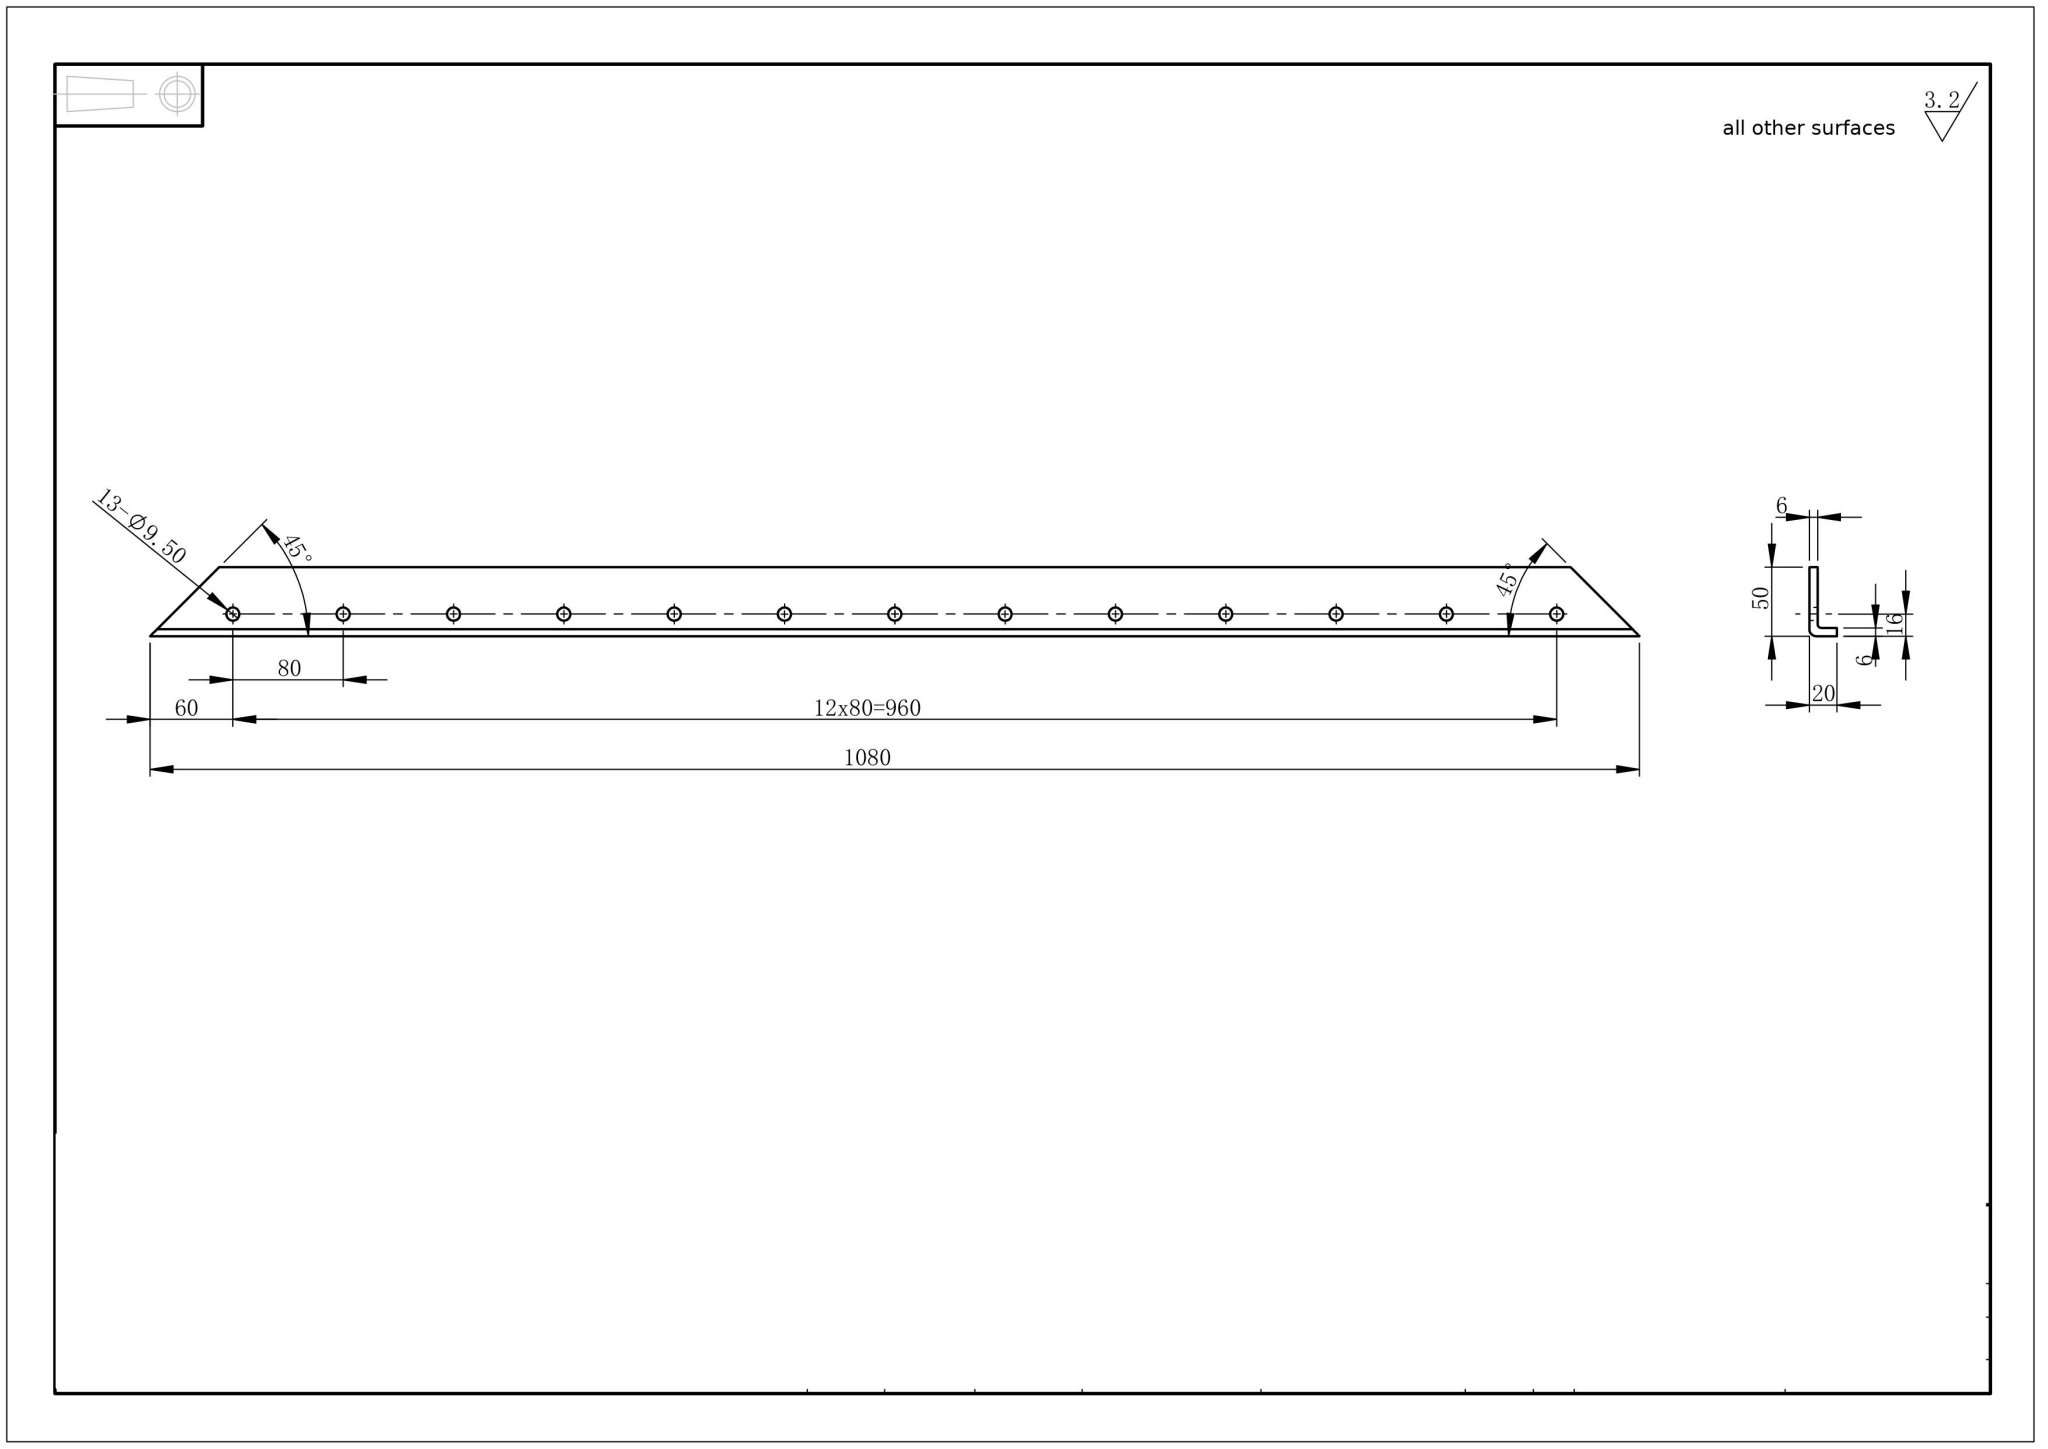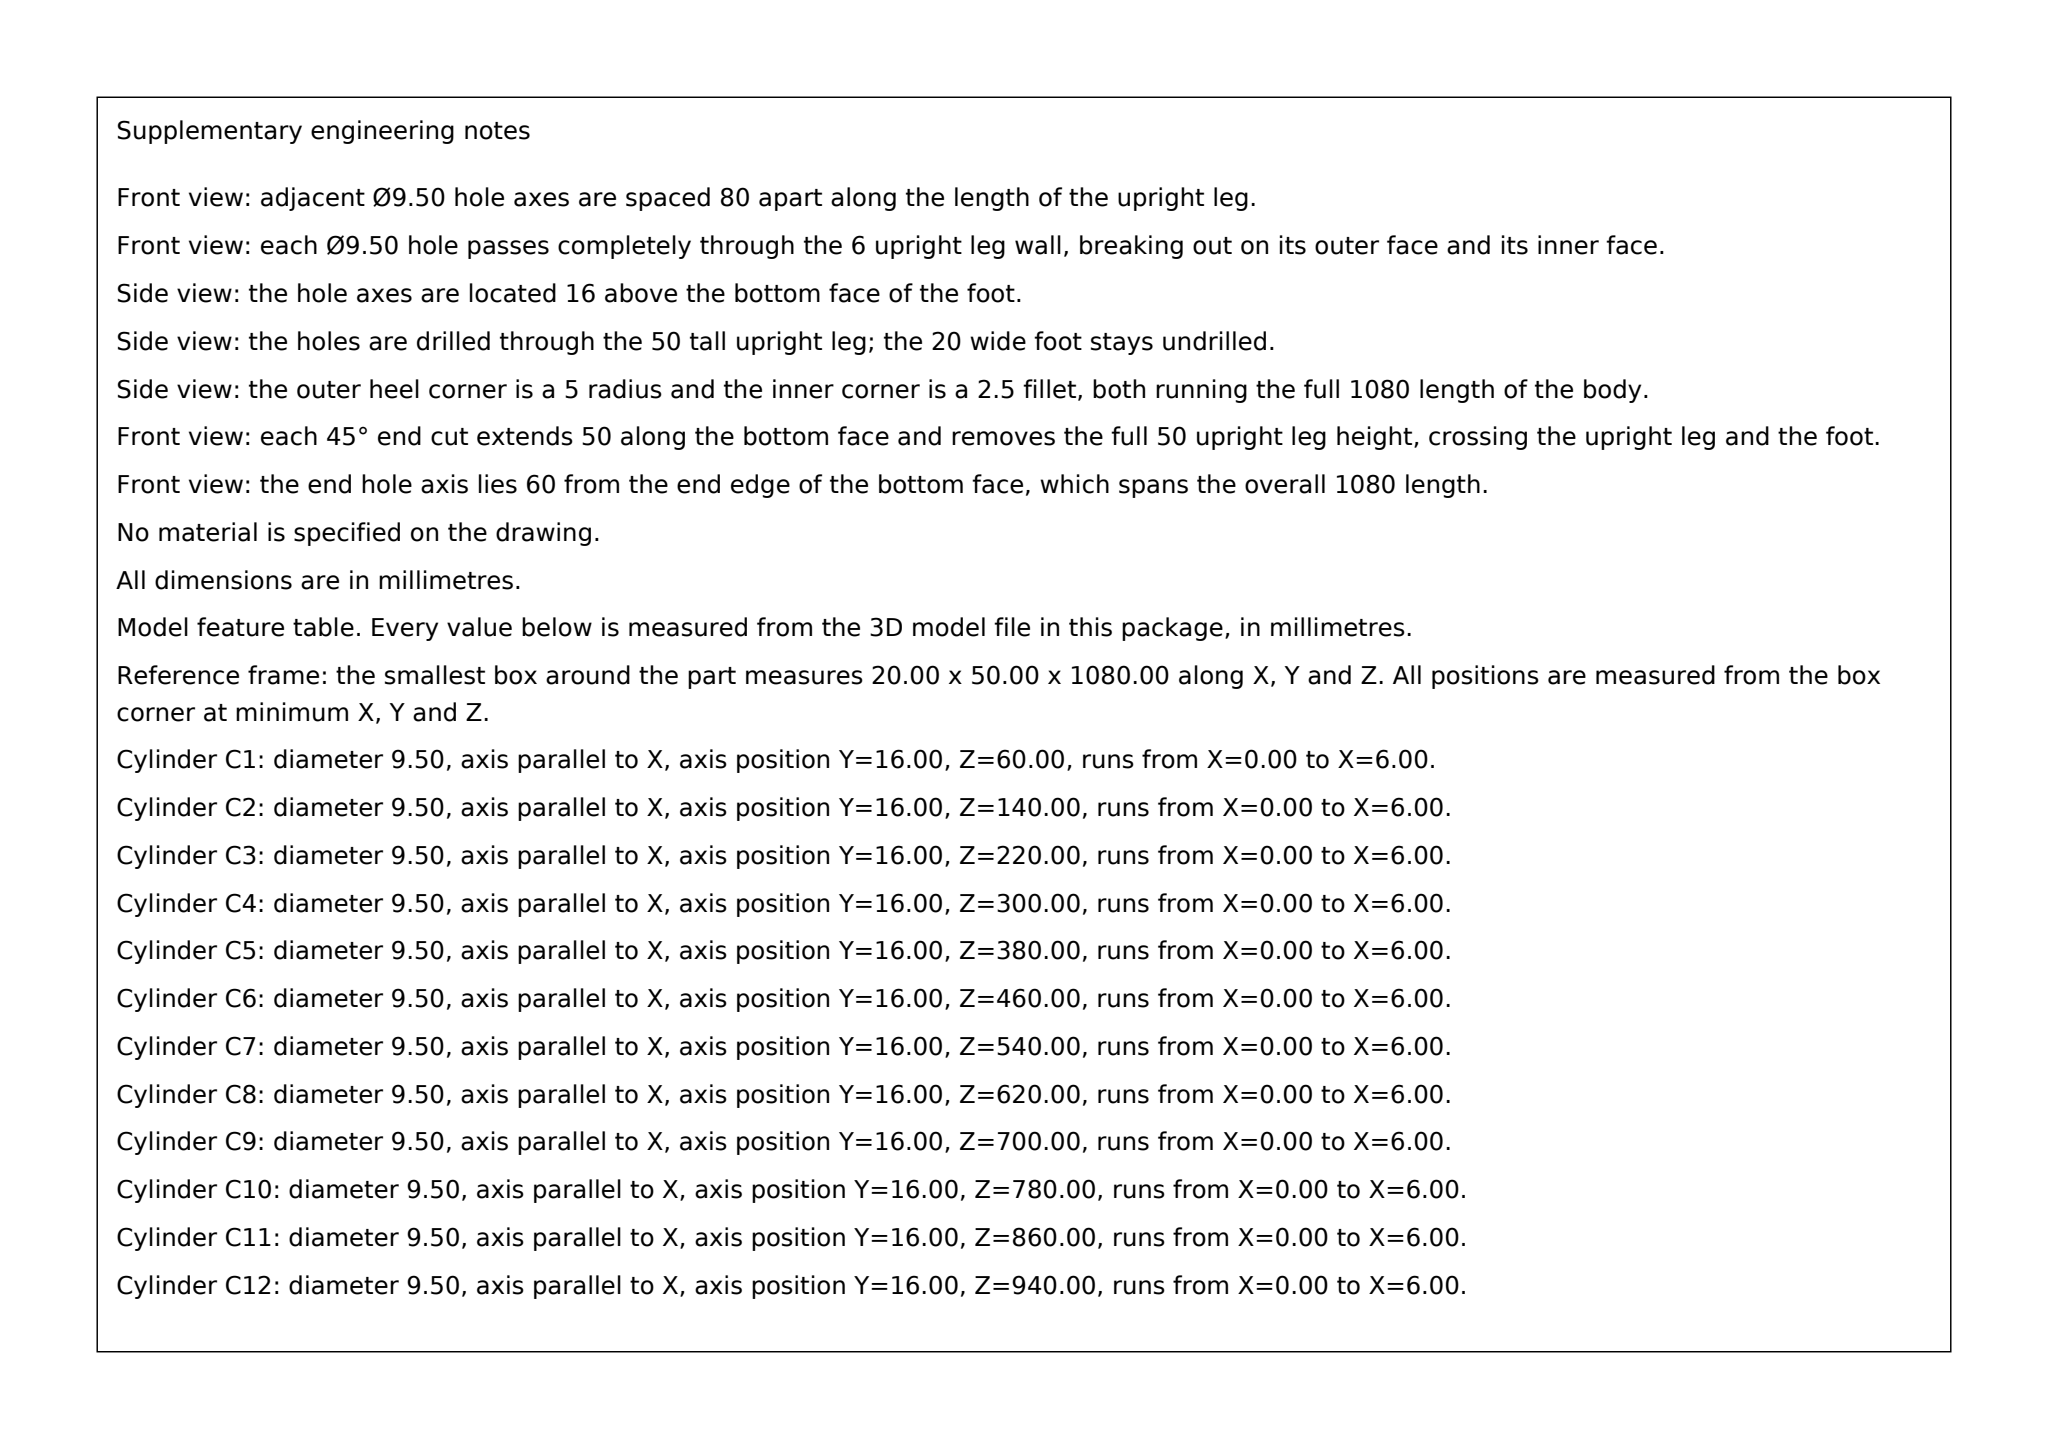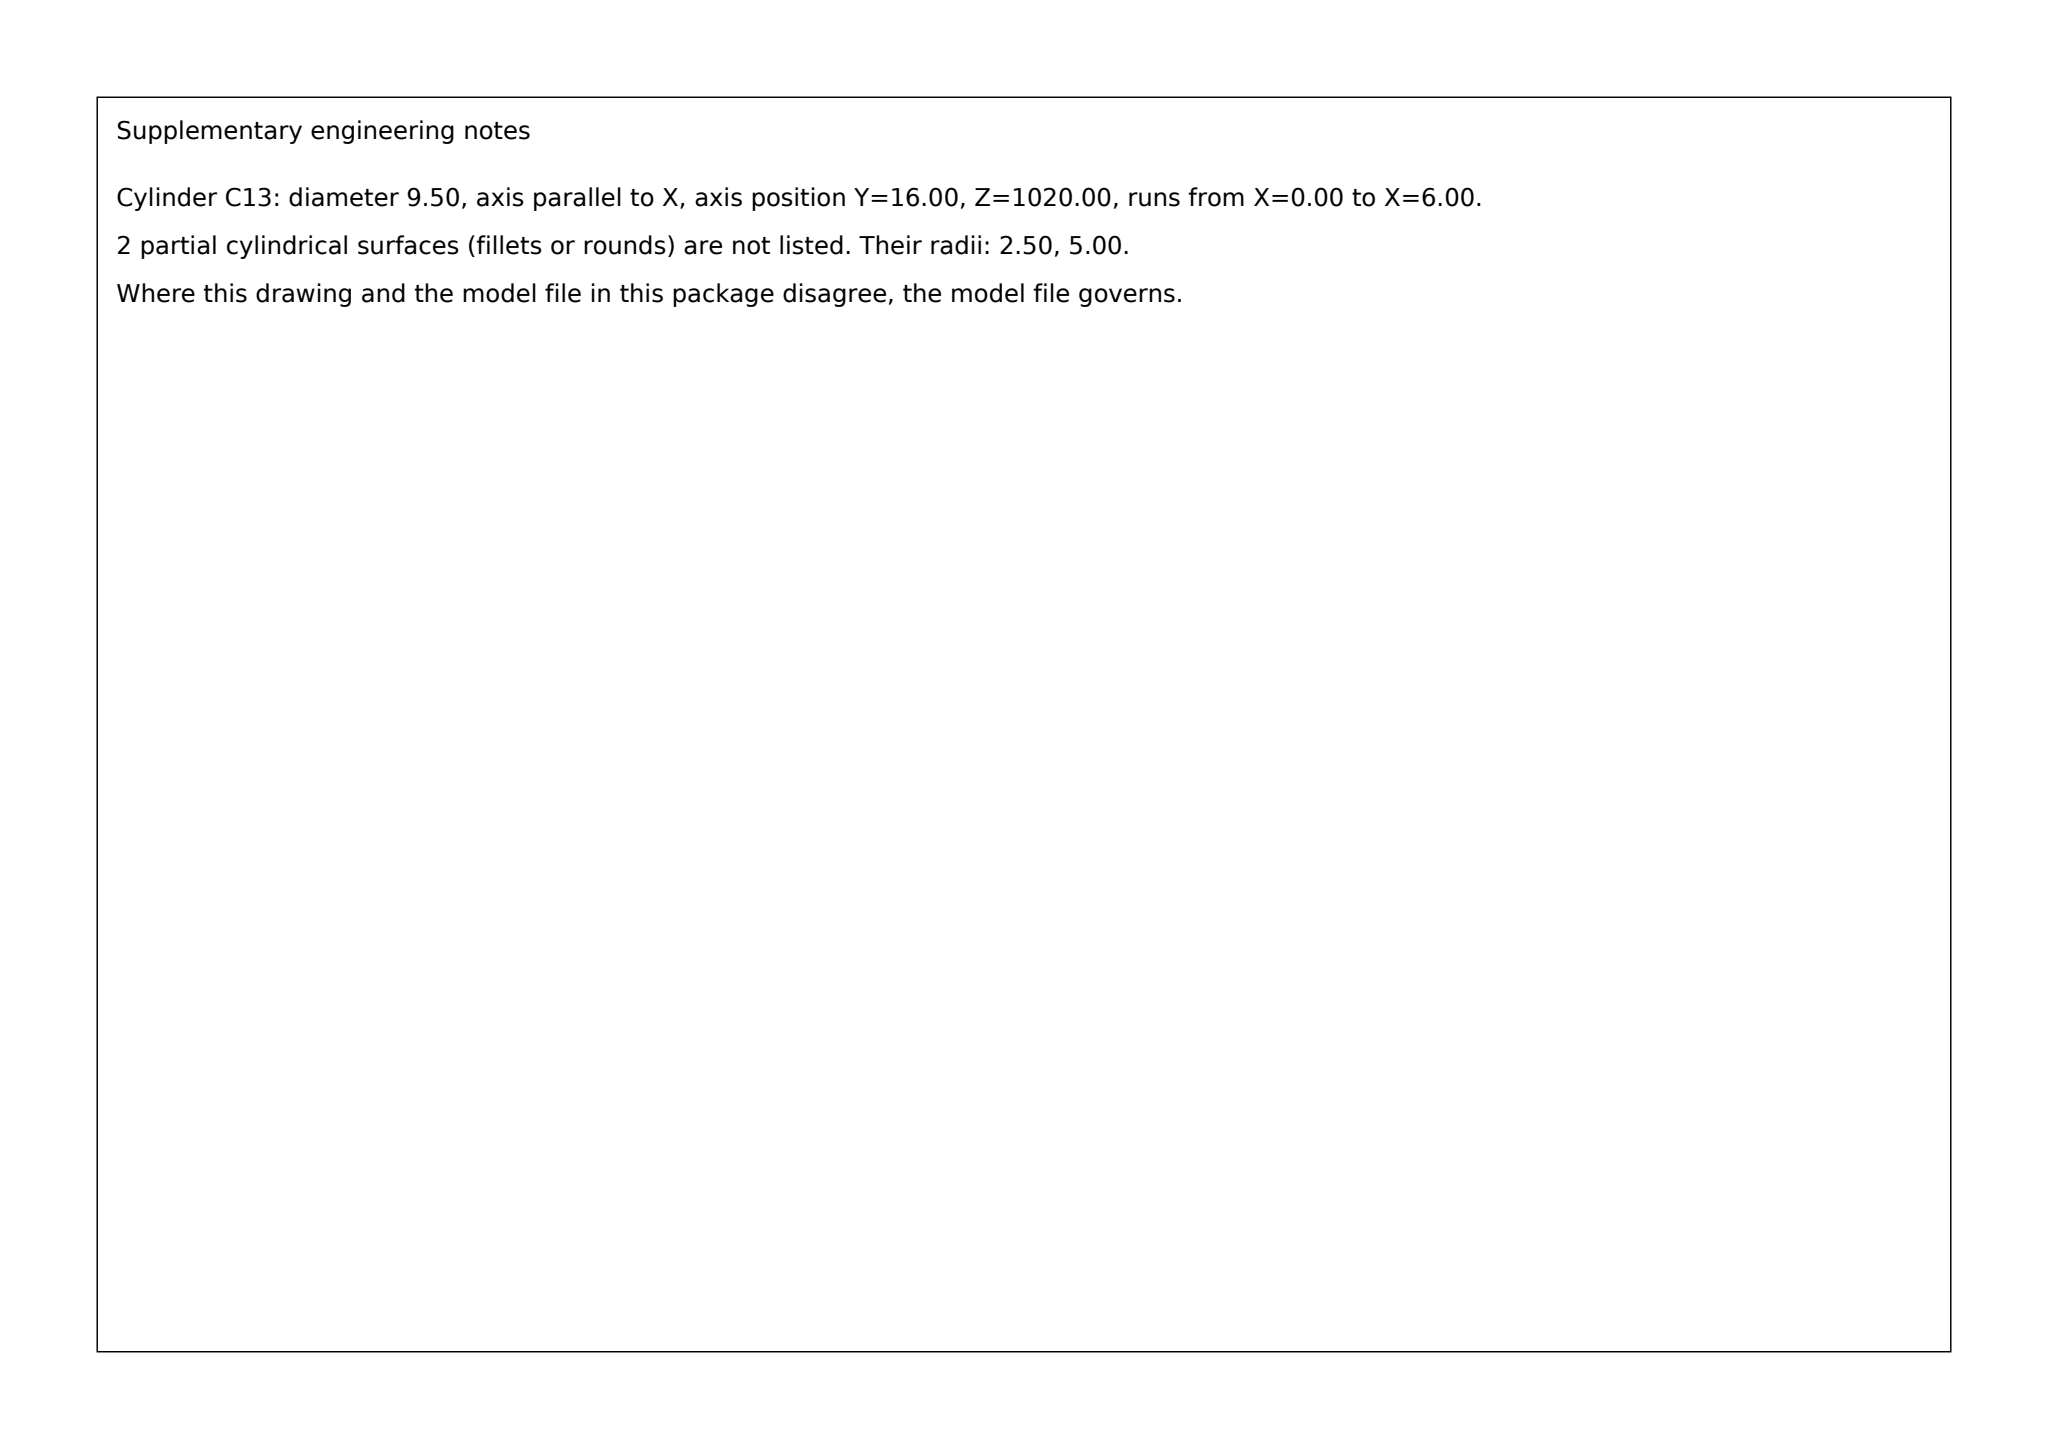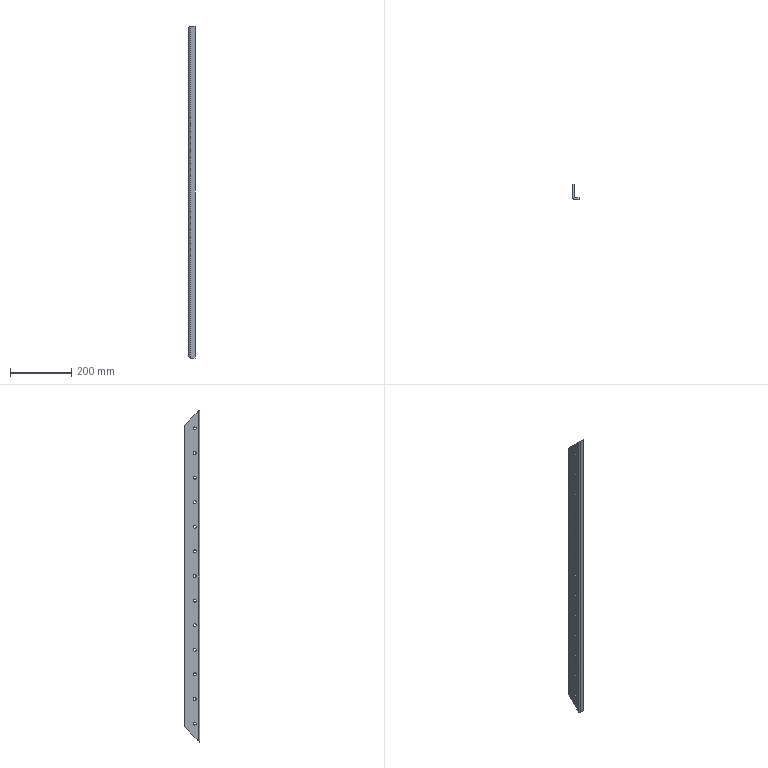Part | SolidWorks | mm | 1 solid | 36 faces | box 20 x 50 x 1080 mm | volume 389336 mm3 | cylinder 28 | plane 8 | commonest cylinder face diameters 9.5 x26 10 x1 5 x1
build123d program:
from build123d import *

# Parameters (mm, degrees)
BOSS_EXTRUDE1_DEPTH        = 1080
CUT_EXTRUDE1_DEPTH         = 1082.342
F_9_5_9_5_DIAMETER_HOLE1_D = 9.5
LPATTERN1_COUNT            = 7
LPATTERN1_PITCH            = 80
LPATTERN2_COUNT            = 7
LPATTERN2_PITCH            = 80


with BuildPart() as part:
    # Sketch1 → Boss-Extrude1 (new body)
    with BuildSketch(Plane.XY):
        with BuildLine():
            Line((-20, 50), (-14, 50))
            Line((-14, 50), (-14, 8.5))
            ThreePointArc((-14, 8.5), (-13.268, 6.732), (-11.5, 6))
            Line((-11.5, 6), (0, 6))
            Line((0, 6), (0, 0))
            Line((0, 0), (-15, 0))
            ThreePointArc((-15, 0), (-18.536, 1.464), (-20, 5))
            Line((-20, 5), (-20, 50))
        make_face()
    extrude(amount=BOSS_EXTRUDE1_DEPTH)

    # Sketch2 → Cut-Extrude1 (cut, through all)
    with BuildSketch(Plane.ZY.offset(20)):
        Polygon((1080, 0), (1030, 50), (1080, 50), align=None)
        Polygon((0, 50), (50, 50), (0, 0), align=None)
    extrude(amount=-CUT_EXTRUDE1_DEPTH, mode=Mode.SUBTRACT)

    # 9.5 _9.5_ Diameter Hole1 (through all)
    with Locations(Plane.ZY.offset(20)):
        with Locations((540, 16)):
            f_9_5_9_5_diameter_hole1 = Hole(F_9_5_9_5_DIAMETER_HOLE1_D / 2)

    # LPattern1: 9.5 _9.5_ Diameter Hole1 ×7
    with Locations(*[(0, 0, -i * LPATTERN1_PITCH) for i in range(1, LPATTERN1_COUNT)]):
        add(f_9_5_9_5_diameter_hole1, mode=Mode.SUBTRACT)

    # LPattern2: 9.5 _9.5_ Diameter Hole1 ×7
    with Locations(*[(0, 0, i * LPATTERN2_PITCH) for i in range(1, LPATTERN2_COUNT)]):
        add(f_9_5_9_5_diameter_hole1, mode=Mode.SUBTRACT)


solid = part.part